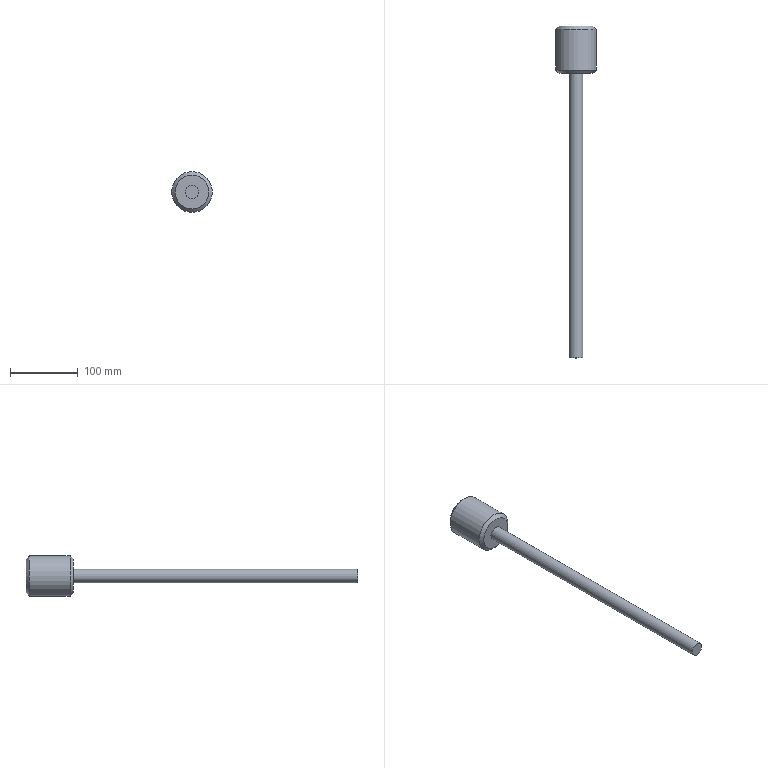Component | NX | EJECTOR1 | 1 solid | 7 faces | box 60 x 490 x 60 mm | volume 325417 mm3 | plane 3 | cylinder 2 | cone 2 | commonest cylinder face diameters 20 x1 60 x1
STEP:
#1=CARTESIAN_POINT('',(0.,0.,0.));
#2=DIRECTION('',(0.,0.,1.));
#3=DIRECTION('',(1.,0.,0.));
#4=AXIS2_PLACEMENT_3D('',#1,#2,#3);
#5=CARTESIAN_POINT('',(10.,117.,0.));
#6=VERTEX_POINT('',#5);
#7=CARTESIAN_POINT('',(-0.,117.,0.));
#8=DIRECTION('',(0.,1.,0.));
#9=DIRECTION('',(1.,0.,0.));
#10=AXIS2_PLACEMENT_3D('',#7,#8,#9);
#11=CIRCLE('',#10,10.);
#12=CARTESIAN_POINT('',(-0.,117.,0.));
#13=DIRECTION('',(0.,-1.,0.));
#14=DIRECTION('',(-1.,0.,0.));
#15=AXIS2_PLACEMENT_3D('',#12,#13,#14);
#16=PLANE('',#15);
#17=CARTESIAN_POINT('',(-10.,0.));
#18=CARTESIAN_POINT('',(-10.,17.321));
#19=CARTESIAN_POINT('',(5.,8.66));
#20=CARTESIAN_POINT('',(20.,0.));
#21=CARTESIAN_POINT('',(5.,-8.66));
#22=CARTESIAN_POINT('',(-10.,-17.321));
#23=CARTESIAN_POINT('',(-10.,0.));
#24=(BOUNDED_CURVE()B_SPLINE_CURVE(2,(#17,#18,#19,#20,#21,#22,#23),.UNSPECIFIED.,.T.,.F.)B_SPLINE_CURVE_WITH_KNOTS((1,2,2,2,2,1),(-2.094,0.,2.094,4.189,6.283,8.378),.UNSPECIFIED.)CURVE()GEOMETRIC_REPRESENTATION_ITEM()RATIONAL_B_SPLINE_CURVE((1.,0.5,1.,0.5,1.,0.5,1.))REPRESENTATION_ITEM(''));
#25=(GEOMETRIC_REPRESENTATION_CONTEXT(2)PARAMETRIC_REPRESENTATION_CONTEXT()REPRESENTATION_CONTEXT('',''));
#26=DEFINITIONAL_REPRESENTATION('',(#24),#25);
#27=PCURVE('',#16,#26);
#28=CARTESIAN_POINT('',(-0.,117.,0.));
#29=DIRECTION('',(0.,1.,0.));
#30=DIRECTION('',(1.,0.,0.));
#31=AXIS2_PLACEMENT_3D('',#28,#29,#30);
#32=CYLINDRICAL_SURFACE('',#31,10.);
#33=CARTESIAN_POINT('',(0.,0.));
#34=DIRECTION('',(1.,0.));
#35=VECTOR('',#34,1.);
#36=LINE('',#33,#35);
#37=(GEOMETRIC_REPRESENTATION_CONTEXT(2)PARAMETRIC_REPRESENTATION_CONTEXT()REPRESENTATION_CONTEXT('',''));
#38=DEFINITIONAL_REPRESENTATION('',(#36),#37);
#39=PCURVE('',#32,#38);
#40=SURFACE_CURVE('',#11,(#27,#39),.PCURVE_S1.);
#41=EDGE_CURVE('',#6,#6,#40,.T.);
#42=ORIENTED_EDGE('',*,*,#41,.F.);
#43=EDGE_LOOP('',(#42));
#44=FACE_BOUND('',#43,.T.);
#45=ADVANCED_FACE('',(#44),#16,.T.);
#46=CARTESIAN_POINT('',(10.,537.,0.));
#47=VERTEX_POINT('',#46);
#48=CARTESIAN_POINT('',(-0.,537.,0.));
#49=DIRECTION('',(0.,-1.,0.));
#50=DIRECTION('',(1.,0.,0.));
#51=AXIS2_PLACEMENT_3D('',#48,#49,#50);
#52=CIRCLE('',#51,10.);
#53=CARTESIAN_POINT('',(6.283,420.));
#54=DIRECTION('',(-1.,0.));
#55=VECTOR('',#54,1.);
#56=LINE('',#53,#55);
#57=(GEOMETRIC_REPRESENTATION_CONTEXT(2)PARAMETRIC_REPRESENTATION_CONTEXT()REPRESENTATION_CONTEXT('',''));
#58=DEFINITIONAL_REPRESENTATION('',(#56),#57);
#59=PCURVE('',#32,#58);
#60=CARTESIAN_POINT('',(-0.,537.,0.));
#61=DIRECTION('',(0.,1.,0.));
#62=DIRECTION('',(1.,0.,0.));
#63=AXIS2_PLACEMENT_3D('',#60,#61,#62);
#64=PLANE('',#63);
#65=CARTESIAN_POINT('',(10.,0.));
#66=CARTESIAN_POINT('',(10.,-17.321));
#67=CARTESIAN_POINT('',(-5.,-8.66));
#68=CARTESIAN_POINT('',(-20.,-0.));
#69=CARTESIAN_POINT('',(-5.,8.66));
#70=CARTESIAN_POINT('',(10.,17.321));
#71=CARTESIAN_POINT('',(10.,0.));
#72=(BOUNDED_CURVE()B_SPLINE_CURVE(2,(#65,#66,#67,#68,#69,#70,#71),.UNSPECIFIED.,.T.,.F.)B_SPLINE_CURVE_WITH_KNOTS((1,2,2,2,2,1),(-2.094,0.,2.094,4.189,6.283,8.378),.UNSPECIFIED.)CURVE()GEOMETRIC_REPRESENTATION_ITEM()RATIONAL_B_SPLINE_CURVE((1.,0.5,1.,0.5,1.,0.5,1.))REPRESENTATION_ITEM(''));
#73=(GEOMETRIC_REPRESENTATION_CONTEXT(2)PARAMETRIC_REPRESENTATION_CONTEXT()REPRESENTATION_CONTEXT('',''));
#74=DEFINITIONAL_REPRESENTATION('',(#72),#73);
#75=PCURVE('',#64,#74);
#76=SURFACE_CURVE('',#52,(#59,#75),.PCURVE_S1.);
#77=EDGE_CURVE('',#47,#47,#76,.T.);
#78=ORIENTED_EDGE('',*,*,#77,.T.);
#79=CARTESIAN_POINT('',(10.,117.,0.));
#80=CARTESIAN_POINT('',(10.,537.,0.));
#81=B_SPLINE_CURVE_WITH_KNOTS('',1,(#79,#80),.UNSPECIFIED.,.F.,.F.,(2,2),(0.,420.),.PIECEWISE_BEZIER_KNOTS.);
#82=CARTESIAN_POINT('',(0.,0.));
#83=DIRECTION('',(0.,1.));
#84=VECTOR('',#83,1.);
#85=LINE('',#82,#84);
#86=(GEOMETRIC_REPRESENTATION_CONTEXT(2)PARAMETRIC_REPRESENTATION_CONTEXT()REPRESENTATION_CONTEXT('',''));
#87=DEFINITIONAL_REPRESENTATION('',(#85),#86);
#88=PCURVE('',#32,#87);
#89=CARTESIAN_POINT('',(6.283,0.));
#90=DIRECTION('',(0.,1.));
#91=VECTOR('',#90,1.);
#92=LINE('',#89,#91);
#93=(GEOMETRIC_REPRESENTATION_CONTEXT(2)PARAMETRIC_REPRESENTATION_CONTEXT()REPRESENTATION_CONTEXT('',''));
#94=DEFINITIONAL_REPRESENTATION('',(#92),#93);
#95=PCURVE('',#32,#94);
#96=SEAM_CURVE('',#81,(#88,#95),.PCURVE_S1.);
#97=EDGE_CURVE('',#6,#47,#96,.T.);
#98=ORIENTED_EDGE('',*,*,#97,.F.);
#99=ORIENTED_EDGE('',*,*,#41,.T.);
#100=ORIENTED_EDGE('',*,*,#97,.T.);
#101=EDGE_LOOP('',(#78,#98,#99,#100));
#102=FACE_BOUND('',#101,.T.);
#103=ADVANCED_FACE('',(#102),#32,.T.);
#104=CARTESIAN_POINT('',(30.,542.,0.));
#105=VERTEX_POINT('',#104);
#106=CARTESIAN_POINT('',(-0.,542.,0.));
#107=DIRECTION('',(0.,1.,0.));
#108=DIRECTION('',(1.,0.,0.));
#109=AXIS2_PLACEMENT_3D('',#106,#107,#108);
#110=CIRCLE('',#109,30.);
#111=CARTESIAN_POINT('',(-0.,607.,0.));
#112=DIRECTION('',(0.,-1.,0.));
#113=DIRECTION('',(-1.,0.,0.));
#114=AXIS2_PLACEMENT_3D('',#111,#112,#113);
#115=CYLINDRICAL_SURFACE('',#114,30.);
#116=CARTESIAN_POINT('',(9.425,65.));
#117=DIRECTION('',(-1.,0.));
#118=VECTOR('',#117,1.);
#119=LINE('',#116,#118);
#120=(GEOMETRIC_REPRESENTATION_CONTEXT(2)PARAMETRIC_REPRESENTATION_CONTEXT()REPRESENTATION_CONTEXT('',''));
#121=DEFINITIONAL_REPRESENTATION('',(#119),#120);
#122=PCURVE('',#115,#121);
#123=CARTESIAN_POINT('',(-0.,542.,0.));
#124=DIRECTION('',(0.,1.,0.));
#125=DIRECTION('',(1.,0.,0.));
#126=AXIS2_PLACEMENT_3D('',#123,#124,#125);
#127=CONICAL_SURFACE('',#126,30.,0.7854);
#128=CARTESIAN_POINT('',(0.,0.));
#129=DIRECTION('',(1.,0.));
#130=VECTOR('',#129,1.);
#131=LINE('',#128,#130);
#132=(GEOMETRIC_REPRESENTATION_CONTEXT(2)PARAMETRIC_REPRESENTATION_CONTEXT()REPRESENTATION_CONTEXT('',''));
#133=DEFINITIONAL_REPRESENTATION('',(#131),#132);
#134=PCURVE('',#127,#133);
#135=SURFACE_CURVE('',#110,(#122,#134),.PCURVE_S1.);
#136=EDGE_CURVE('',#105,#105,#135,.T.);
#137=ORIENTED_EDGE('',*,*,#136,.T.);
#138=CARTESIAN_POINT('',(30.,602.,0.));
#139=VERTEX_POINT('',#138);
#140=CARTESIAN_POINT('',(30.,602.,0.));
#141=CARTESIAN_POINT('',(30.,542.,0.));
#142=B_SPLINE_CURVE_WITH_KNOTS('',1,(#140,#141),.UNSPECIFIED.,.F.,.F.,(2,2),(5.,65.),.PIECEWISE_BEZIER_KNOTS.);
#143=CARTESIAN_POINT('',(3.142,0.));
#144=DIRECTION('',(0.,1.));
#145=VECTOR('',#144,1.);
#146=LINE('',#143,#145);
#147=(GEOMETRIC_REPRESENTATION_CONTEXT(2)PARAMETRIC_REPRESENTATION_CONTEXT()REPRESENTATION_CONTEXT('',''));
#148=DEFINITIONAL_REPRESENTATION('',(#146),#147);
#149=PCURVE('',#115,#148);
#150=CARTESIAN_POINT('',(9.425,0.));
#151=DIRECTION('',(0.,1.));
#152=VECTOR('',#151,1.);
#153=LINE('',#150,#152);
#154=(GEOMETRIC_REPRESENTATION_CONTEXT(2)PARAMETRIC_REPRESENTATION_CONTEXT()REPRESENTATION_CONTEXT('',''));
#155=DEFINITIONAL_REPRESENTATION('',(#153),#154);
#156=PCURVE('',#115,#155);
#157=SEAM_CURVE('',#142,(#149,#156),.PCURVE_S1.);
#158=EDGE_CURVE('',#139,#105,#157,.T.);
#159=ORIENTED_EDGE('',*,*,#158,.F.);
#160=CARTESIAN_POINT('',(-0.,602.,0.));
#161=DIRECTION('',(0.,-1.,0.));
#162=DIRECTION('',(1.,0.,0.));
#163=AXIS2_PLACEMENT_3D('',#160,#161,#162);
#164=CIRCLE('',#163,30.);
#165=CARTESIAN_POINT('',(3.142,5.));
#166=DIRECTION('',(1.,0.));
#167=VECTOR('',#166,1.);
#168=LINE('',#165,#167);
#169=(GEOMETRIC_REPRESENTATION_CONTEXT(2)PARAMETRIC_REPRESENTATION_CONTEXT()REPRESENTATION_CONTEXT('',''));
#170=DEFINITIONAL_REPRESENTATION('',(#168),#169);
#171=PCURVE('',#115,#170);
#172=CARTESIAN_POINT('',(-0.,607.,0.));
#173=DIRECTION('',(0.,-1.,0.));
#174=DIRECTION('',(-1.,0.,0.));
#175=AXIS2_PLACEMENT_3D('',#172,#173,#174);
#176=CONICAL_SURFACE('',#175,25.,0.7854);
#177=CARTESIAN_POINT('',(3.142,5.));
#178=DIRECTION('',(1.,0.));
#179=VECTOR('',#178,1.);
#180=LINE('',#177,#179);
#181=(GEOMETRIC_REPRESENTATION_CONTEXT(2)PARAMETRIC_REPRESENTATION_CONTEXT()REPRESENTATION_CONTEXT('',''));
#182=DEFINITIONAL_REPRESENTATION('',(#180),#181);
#183=PCURVE('',#176,#182);
#184=SURFACE_CURVE('',#164,(#171,#183),.PCURVE_S1.);
#185=EDGE_CURVE('',#139,#139,#184,.T.);
#186=ORIENTED_EDGE('',*,*,#185,.T.);
#187=ORIENTED_EDGE('',*,*,#158,.T.);
#188=EDGE_LOOP('',(#137,#159,#186,#187));
#189=FACE_BOUND('',#188,.T.);
#190=ADVANCED_FACE('',(#189),#115,.T.);
#191=CARTESIAN_POINT('',(25.,607.,0.));
#192=VERTEX_POINT('',#191);
#193=CARTESIAN_POINT('',(-0.,607.,0.));
#194=DIRECTION('',(0.,1.,0.));
#195=DIRECTION('',(1.,0.,0.));
#196=AXIS2_PLACEMENT_3D('',#193,#194,#195);
#197=CIRCLE('',#196,25.);
#198=CARTESIAN_POINT('',(-0.,607.,0.));
#199=DIRECTION('',(0.,1.,0.));
#200=DIRECTION('',(1.,0.,0.));
#201=AXIS2_PLACEMENT_3D('',#198,#199,#200);
#202=PLANE('',#201);
#203=CARTESIAN_POINT('',(0.,0.));
#204=DIRECTION('',(1.,0.));
#205=AXIS2_PLACEMENT_2D('',#203,#204);
#206=CIRCLE('',#205,25.);
#207=(GEOMETRIC_REPRESENTATION_CONTEXT(2)PARAMETRIC_REPRESENTATION_CONTEXT()REPRESENTATION_CONTEXT('',''));
#208=DEFINITIONAL_REPRESENTATION('',(#206),#207);
#209=PCURVE('',#202,#208);
#210=CARTESIAN_POINT('',(9.425,0.));
#211=DIRECTION('',(-1.,0.));
#212=VECTOR('',#211,1.);
#213=LINE('',#210,#212);
#214=(GEOMETRIC_REPRESENTATION_CONTEXT(2)PARAMETRIC_REPRESENTATION_CONTEXT()REPRESENTATION_CONTEXT('',''));
#215=DEFINITIONAL_REPRESENTATION('',(#213),#214);
#216=PCURVE('',#176,#215);
#217=SURFACE_CURVE('',#197,(#209,#216),.PCURVE_S1.);
#218=EDGE_CURVE('',#192,#192,#217,.T.);
#219=ORIENTED_EDGE('',*,*,#218,.T.);
#220=EDGE_LOOP('',(#219));
#221=FACE_BOUND('',#220,.T.);
#222=ADVANCED_FACE('',(#221),#202,.T.);
#223=CARTESIAN_POINT('',(25.,537.,0.));
#224=VERTEX_POINT('',#223);
#225=CARTESIAN_POINT('',(-0.,537.,0.));
#226=DIRECTION('',(0.,-1.,0.));
#227=DIRECTION('',(1.,0.,0.));
#228=AXIS2_PLACEMENT_3D('',#225,#226,#227);
#229=CIRCLE('',#228,25.);
#230=CARTESIAN_POINT('',(25.,0.));
#231=CARTESIAN_POINT('',(25.,-43.301));
#232=CARTESIAN_POINT('',(-12.5,-21.651));
#233=CARTESIAN_POINT('',(-50.,-0.));
#234=CARTESIAN_POINT('',(-12.5,21.651));
#235=CARTESIAN_POINT('',(25.,43.301));
#236=CARTESIAN_POINT('',(25.,0.));
#237=(BOUNDED_CURVE()B_SPLINE_CURVE(2,(#230,#231,#232,#233,#234,#235,#236),.UNSPECIFIED.,.T.,.F.)B_SPLINE_CURVE_WITH_KNOTS((1,2,2,2,2,1),(-2.094,0.,2.094,4.189,6.283,8.378),.UNSPECIFIED.)CURVE()GEOMETRIC_REPRESENTATION_ITEM()RATIONAL_B_SPLINE_CURVE((1.,0.5,1.,0.5,1.,0.5,1.))REPRESENTATION_ITEM(''));
#238=(GEOMETRIC_REPRESENTATION_CONTEXT(2)PARAMETRIC_REPRESENTATION_CONTEXT()REPRESENTATION_CONTEXT('',''));
#239=DEFINITIONAL_REPRESENTATION('',(#237),#238);
#240=PCURVE('',#64,#239);
#241=CARTESIAN_POINT('',(6.283,-5.));
#242=DIRECTION('',(-1.,0.));
#243=VECTOR('',#242,1.);
#244=LINE('',#241,#243);
#245=(GEOMETRIC_REPRESENTATION_CONTEXT(2)PARAMETRIC_REPRESENTATION_CONTEXT()REPRESENTATION_CONTEXT('',''));
#246=DEFINITIONAL_REPRESENTATION('',(#244),#245);
#247=PCURVE('',#127,#246);
#248=SURFACE_CURVE('',#229,(#240,#247),.PCURVE_S1.);
#249=EDGE_CURVE('',#224,#224,#248,.T.);
#250=ORIENTED_EDGE('',*,*,#249,.T.);
#251=EDGE_LOOP('',(#250));
#252=FACE_BOUND('',#251,.T.);
#253=ORIENTED_EDGE('',*,*,#77,.F.);
#254=EDGE_LOOP('',(#253));
#255=FACE_BOUND('',#254,.T.);
#256=ADVANCED_FACE('',(#252,#255),#64,.F.);
#257=ORIENTED_EDGE('',*,*,#249,.F.);
#258=CARTESIAN_POINT('',(25.,537.,0.));
#259=CARTESIAN_POINT('',(30.,542.,0.));
#260=B_SPLINE_CURVE_WITH_KNOTS('',1,(#258,#259),.UNSPECIFIED.,.F.,.F.,(2,2),(-7.071,0.),.PIECEWISE_BEZIER_KNOTS.);
#261=CARTESIAN_POINT('',(6.283,0.));
#262=DIRECTION('',(0.,1.));
#263=VECTOR('',#262,1.);
#264=LINE('',#261,#263);
#265=(GEOMETRIC_REPRESENTATION_CONTEXT(2)PARAMETRIC_REPRESENTATION_CONTEXT()REPRESENTATION_CONTEXT('',''));
#266=DEFINITIONAL_REPRESENTATION('',(#264),#265);
#267=PCURVE('',#127,#266);
#268=CARTESIAN_POINT('',(0.,0.));
#269=DIRECTION('',(0.,1.));
#270=VECTOR('',#269,1.);
#271=LINE('',#268,#270);
#272=(GEOMETRIC_REPRESENTATION_CONTEXT(2)PARAMETRIC_REPRESENTATION_CONTEXT()REPRESENTATION_CONTEXT('',''));
#273=DEFINITIONAL_REPRESENTATION('',(#271),#272);
#274=PCURVE('',#127,#273);
#275=SEAM_CURVE('',#260,(#267,#274),.PCURVE_S1.);
#276=EDGE_CURVE('',#224,#105,#275,.T.);
#277=ORIENTED_EDGE('',*,*,#276,.T.);
#278=ORIENTED_EDGE('',*,*,#136,.F.);
#279=ORIENTED_EDGE('',*,*,#276,.F.);
#280=EDGE_LOOP('',(#257,#277,#278,#279));
#281=FACE_BOUND('',#280,.T.);
#282=ADVANCED_FACE('',(#281),#127,.T.);
#283=ORIENTED_EDGE('',*,*,#185,.F.);
#284=CARTESIAN_POINT('',(25.,607.,0.));
#285=CARTESIAN_POINT('',(30.,602.,0.));
#286=B_SPLINE_CURVE_WITH_KNOTS('',1,(#284,#285),.UNSPECIFIED.,.F.,.F.,(2,2),(0.,7.071),.PIECEWISE_BEZIER_KNOTS.);
#287=CARTESIAN_POINT('',(3.142,0.));
#288=DIRECTION('',(0.,1.));
#289=VECTOR('',#288,1.);
#290=LINE('',#287,#289);
#291=(GEOMETRIC_REPRESENTATION_CONTEXT(2)PARAMETRIC_REPRESENTATION_CONTEXT()REPRESENTATION_CONTEXT('',''));
#292=DEFINITIONAL_REPRESENTATION('',(#290),#291);
#293=PCURVE('',#176,#292);
#294=CARTESIAN_POINT('',(9.425,0.));
#295=DIRECTION('',(0.,1.));
#296=VECTOR('',#295,1.);
#297=LINE('',#294,#296);
#298=(GEOMETRIC_REPRESENTATION_CONTEXT(2)PARAMETRIC_REPRESENTATION_CONTEXT()REPRESENTATION_CONTEXT('',''));
#299=DEFINITIONAL_REPRESENTATION('',(#297),#298);
#300=PCURVE('',#176,#299);
#301=SEAM_CURVE('',#286,(#293,#300),.PCURVE_S1.);
#302=EDGE_CURVE('',#192,#139,#301,.T.);
#303=ORIENTED_EDGE('',*,*,#302,.F.);
#304=ORIENTED_EDGE('',*,*,#218,.F.);
#305=ORIENTED_EDGE('',*,*,#302,.T.);
#306=EDGE_LOOP('',(#283,#303,#304,#305));
#307=FACE_BOUND('',#306,.T.);
#308=ADVANCED_FACE('',(#307),#176,.T.);
#309=CLOSED_SHELL('',(#45,#103,#190,#222,#256,#282,#308));
#310=MANIFOLD_SOLID_BREP('',#309);
#311=(LENGTH_UNIT()NAMED_UNIT(*)SI_UNIT(.MILLI.,.METRE.));
#312=UNCERTAINTY_MEASURE_WITH_UNIT(LENGTH_MEASURE(0.00001),#311,'','');
#313=(NAMED_UNIT(*)PLANE_ANGLE_UNIT()SI_UNIT($,.RADIAN.));
#314=(NAMED_UNIT(*)SI_UNIT($,.STERADIAN.)SOLID_ANGLE_UNIT());
#315=(GEOMETRIC_REPRESENTATION_CONTEXT(3)GLOBAL_UNCERTAINTY_ASSIGNED_CONTEXT((#312))GLOBAL_UNIT_ASSIGNED_CONTEXT((#311,#313,#314))REPRESENTATION_CONTEXT('',''));
#316=ADVANCED_BREP_SHAPE_REPRESENTATION('',(#4,#310),#315);